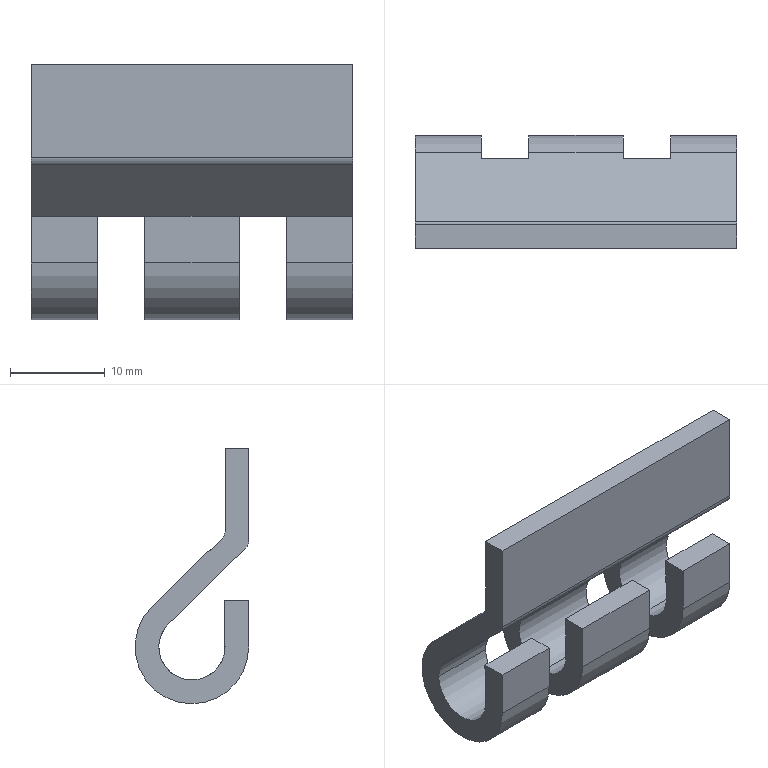Component | SolidWorks | FrontDoorAssembly-1_FrontDoorWelding-1_CL20-1Hinge(1)-1 | 1 solid | 37 faces | volume 3155 mm3 | plane 22 | cylinder 15 | commonest cylinder face diameters 7 x7 12 x6 2 x2